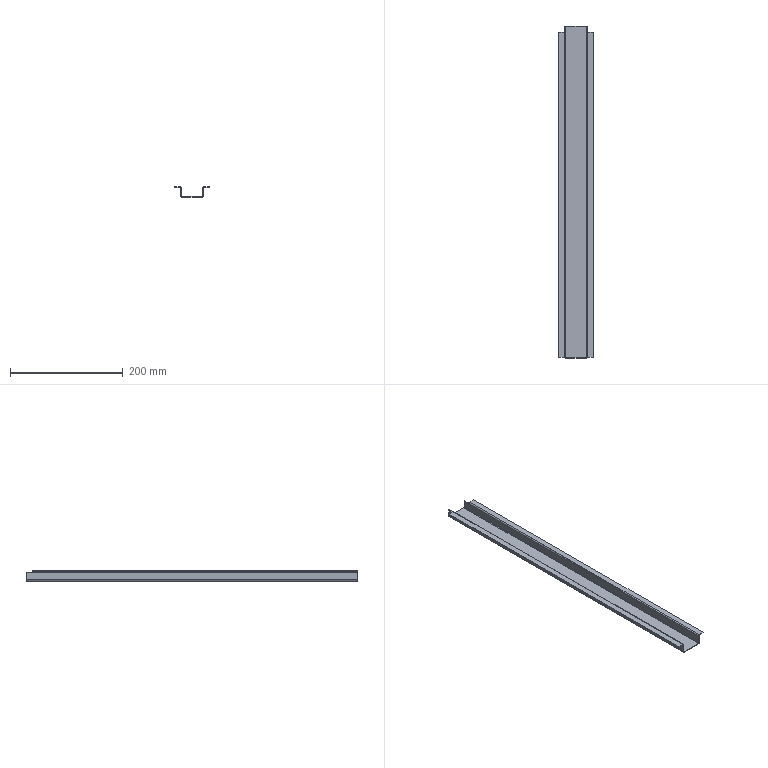Component | SolidWorks | AirFurnaceElectricalCabinet-DoorPanelAssembly-1_DoorPanelReinforcementPlate-L590-1 | 1 solid | 38 faces | box 61.6 x 590 x 18 mm | volume 65385 mm3 | plane 30 | cylinder 8 | commonest cylinder face diameters 3.9 x4 1.5 x4
STEP:
#1=COLOUR_RGB('',0.7922,0.8196,0.9333);
#2=FILL_AREA_STYLE_COLOUR('',#1);
#3=FILL_AREA_STYLE('',(#2));
#4=SURFACE_STYLE_FILL_AREA(#3);
#5=SURFACE_SIDE_STYLE('',(#4));
#6=SURFACE_STYLE_USAGE(.BOTH.,#5);
#7=PRESENTATION_STYLE_ASSIGNMENT((#6));
#8=CARTESIAN_POINT('',(0.7402,27.303,9.348));
#9=VERTEX_POINT('',#8);
#10=CARTESIAN_POINT('',(0.7402,27.303,9.882));
#11=VERTEX_POINT('',#10);
#12=CARTESIAN_POINT('',(0.7402,27.303,9.272));
#13=DIRECTION('',(-0.,-0.,1.));
#14=VECTOR('',#13,39.37);
#15=LINE('',#12,#14);
#16=EDGE_CURVE('',#9,#11,#15,.T.);
#17=ORIENTED_EDGE('',*,*,#16,.T.);
#18=CARTESIAN_POINT('',(0.7874,27.303,9.882));
#19=VERTEX_POINT('',#18);
#20=CARTESIAN_POINT('',(0.7106,27.303,9.882));
#21=DIRECTION('',(1.,-0.,0.));
#22=VECTOR('',#21,39.37);
#23=LINE('',#20,#22);
#24=EDGE_CURVE('',#11,#19,#23,.T.);
#25=ORIENTED_EDGE('',*,*,#24,.T.);
#26=CARTESIAN_POINT('',(0.7874,27.303,9.348));
#27=VERTEX_POINT('',#26);
#28=CARTESIAN_POINT('',(0.7874,27.303,9.272));
#29=DIRECTION('',(-0.,-0.,1.));
#30=VECTOR('',#29,39.37);
#31=LINE('',#28,#30);
#32=EDGE_CURVE('',#27,#19,#31,.T.);
#33=ORIENTED_EDGE('',*,*,#32,.F.);
#34=CARTESIAN_POINT('',(0.7874,27.303,9.348));
#35=DIRECTION('',(-1.,0.,-0.));
#36=VECTOR('',#35,39.37);
#37=LINE('',#34,#36);
#38=EDGE_CURVE('',#27,#9,#37,.T.);
#39=ORIENTED_EDGE('',*,*,#38,.T.);
#40=EDGE_LOOP('',(#17,#25,#33,#39));
#41=FACE_OUTER_BOUND('',#40,.T.);
#42=CARTESIAN_POINT('',(0.7106,27.303,9.319));
#43=DIRECTION('',(0.,1.,0.));
#44=DIRECTION('',(1.,-0.,0.));
#45=AXIS2_PLACEMENT_3D('',#42,#43,#44);
#46=PLANE('',#45);
#47=ADVANCED_FACE('',(#41),#46,.T.);
#48=CARTESIAN_POINT('',(0.7874,4.075,9.348));
#49=VERTEX_POINT('',#48);
#50=CARTESIAN_POINT('',(0.7874,4.075,9.882));
#51=VERTEX_POINT('',#50);
#52=CARTESIAN_POINT('',(0.7874,4.075,9.272));
#53=DIRECTION('',(-0.,-0.,1.));
#54=VECTOR('',#53,39.37);
#55=LINE('',#52,#54);
#56=EDGE_CURVE('',#49,#51,#55,.T.);
#57=ORIENTED_EDGE('',*,*,#56,.T.);
#58=CARTESIAN_POINT('',(0.7402,4.075,9.882));
#59=VERTEX_POINT('',#58);
#60=CARTESIAN_POINT('',(0.8169,4.075,9.882));
#61=DIRECTION('',(-1.,0.,-0.));
#62=VECTOR('',#61,39.37);
#63=LINE('',#60,#62);
#64=EDGE_CURVE('',#51,#59,#63,.T.);
#65=ORIENTED_EDGE('',*,*,#64,.T.);
#66=CARTESIAN_POINT('',(0.7402,4.075,9.348));
#67=VERTEX_POINT('',#66);
#68=CARTESIAN_POINT('',(0.7402,4.075,9.272));
#69=DIRECTION('',(-0.,-0.,1.));
#70=VECTOR('',#69,39.37);
#71=LINE('',#68,#70);
#72=EDGE_CURVE('',#67,#59,#71,.T.);
#73=ORIENTED_EDGE('',*,*,#72,.F.);
#74=CARTESIAN_POINT('',(0.7402,4.075,9.348));
#75=DIRECTION('',(1.,-0.,0.));
#76=VECTOR('',#75,39.37);
#77=LINE('',#74,#76);
#78=EDGE_CURVE('',#67,#49,#77,.T.);
#79=ORIENTED_EDGE('',*,*,#78,.T.);
#80=EDGE_LOOP('',(#57,#65,#73,#79));
#81=FACE_OUTER_BOUND('',#80,.T.);
#82=CARTESIAN_POINT('',(0.8169,4.075,9.98));
#83=DIRECTION('',(-0.,-1.,-0.));
#84=DIRECTION('',(-1.,0.,-0.));
#85=AXIS2_PLACEMENT_3D('',#82,#83,#84);
#86=PLANE('',#85);
#87=ADVANCED_FACE('',(#81),#86,.T.);
#88=CARTESIAN_POINT('',(-0.7402,4.075,9.882));
#89=VERTEX_POINT('',#88);
#90=CARTESIAN_POINT('',(-0.7402,4.075,9.348));
#91=VERTEX_POINT('',#90);
#92=CARTESIAN_POINT('',(-0.7402,4.075,9.933));
#93=DIRECTION('',(0.,0.,-1.));
#94=VECTOR('',#93,39.37);
#95=LINE('',#92,#94);
#96=EDGE_CURVE('',#89,#91,#95,.T.);
#97=ORIENTED_EDGE('',*,*,#96,.F.);
#98=CARTESIAN_POINT('',(-0.7874,4.075,9.882));
#99=VERTEX_POINT('',#98);
#100=CARTESIAN_POINT('',(-0.7106,4.075,9.882));
#101=DIRECTION('',(-1.,0.,-0.));
#102=VECTOR('',#101,39.37);
#103=LINE('',#100,#102);
#104=EDGE_CURVE('',#89,#99,#103,.T.);
#105=ORIENTED_EDGE('',*,*,#104,.T.);
#106=CARTESIAN_POINT('',(-0.7874,4.075,9.348));
#107=VERTEX_POINT('',#106);
#108=CARTESIAN_POINT('',(-0.7874,4.075,9.933));
#109=DIRECTION('',(0.,0.,-1.));
#110=VECTOR('',#109,39.37);
#111=LINE('',#108,#110);
#112=EDGE_CURVE('',#99,#107,#111,.T.);
#113=ORIENTED_EDGE('',*,*,#112,.T.);
#114=CARTESIAN_POINT('',(-0.7874,4.075,9.348));
#115=DIRECTION('',(1.,-0.,0.));
#116=VECTOR('',#115,39.37);
#117=LINE('',#114,#116);
#118=EDGE_CURVE('',#107,#91,#117,.T.);
#119=ORIENTED_EDGE('',*,*,#118,.T.);
#120=EDGE_LOOP('',(#97,#105,#113,#119));
#121=FACE_OUTER_BOUND('',#120,.T.);
#122=CARTESIAN_POINT('',(-0.7106,4.075,9.319));
#123=DIRECTION('',(-0.,-1.,-0.));
#124=DIRECTION('',(-1.,0.,-0.));
#125=AXIS2_PLACEMENT_3D('',#122,#123,#124);
#126=PLANE('',#125);
#127=ADVANCED_FACE('',(#121),#126,.T.);
#128=CARTESIAN_POINT('',(-0.7874,27.303,9.882));
#129=VERTEX_POINT('',#128);
#130=CARTESIAN_POINT('',(-0.7874,27.303,9.348));
#131=VERTEX_POINT('',#130);
#132=CARTESIAN_POINT('',(-0.7874,27.303,9.933));
#133=DIRECTION('',(0.,0.,-1.));
#134=VECTOR('',#133,39.37);
#135=LINE('',#132,#134);
#136=EDGE_CURVE('',#129,#131,#135,.T.);
#137=ORIENTED_EDGE('',*,*,#136,.F.);
#138=CARTESIAN_POINT('',(-0.7402,27.303,9.882));
#139=VERTEX_POINT('',#138);
#140=CARTESIAN_POINT('',(-0.8169,27.303,9.882));
#141=DIRECTION('',(1.,-0.,0.));
#142=VECTOR('',#141,39.37);
#143=LINE('',#140,#142);
#144=EDGE_CURVE('',#129,#139,#143,.T.);
#145=ORIENTED_EDGE('',*,*,#144,.T.);
#146=CARTESIAN_POINT('',(-0.7402,27.303,9.348));
#147=VERTEX_POINT('',#146);
#148=CARTESIAN_POINT('',(-0.7402,27.303,9.933));
#149=DIRECTION('',(0.,0.,-1.));
#150=VECTOR('',#149,39.37);
#151=LINE('',#148,#150);
#152=EDGE_CURVE('',#139,#147,#151,.T.);
#153=ORIENTED_EDGE('',*,*,#152,.T.);
#154=CARTESIAN_POINT('',(-0.7402,27.303,9.348));
#155=DIRECTION('',(-1.,0.,-0.));
#156=VECTOR('',#155,39.37);
#157=LINE('',#154,#156);
#158=EDGE_CURVE('',#147,#131,#157,.T.);
#159=ORIENTED_EDGE('',*,*,#158,.T.);
#160=EDGE_LOOP('',(#137,#145,#153,#159));
#161=FACE_OUTER_BOUND('',#160,.T.);
#162=CARTESIAN_POINT('',(-0.8169,27.303,9.98));
#163=DIRECTION('',(0.,1.,0.));
#164=DIRECTION('',(1.,-0.,0.));
#165=AXIS2_PLACEMENT_3D('',#162,#163,#164);
#166=PLANE('',#165);
#167=ADVANCED_FACE('',(#161),#166,.T.);
#168=CARTESIAN_POINT('',(-0.7106,27.303,9.272));
#169=VERTEX_POINT('',#168);
#170=CARTESIAN_POINT('',(0.7106,27.303,9.272));
#171=VERTEX_POINT('',#170);
#172=CARTESIAN_POINT('',(-0.7874,27.303,9.272));
#173=DIRECTION('',(1.,-0.,0.));
#174=VECTOR('',#173,39.37);
#175=LINE('',#172,#174);
#176=EDGE_CURVE('',#169,#171,#175,.T.);
#177=ORIENTED_EDGE('',*,*,#176,.F.);
#178=CARTESIAN_POINT('',(-0.7106,27.303,9.319));
#179=VERTEX_POINT('',#178);
#180=CARTESIAN_POINT('',(-0.7106,27.303,9.272));
#181=DIRECTION('',(-0.,-0.,1.));
#182=VECTOR('',#181,39.37);
#183=LINE('',#180,#182);
#184=EDGE_CURVE('',#169,#179,#183,.T.);
#185=ORIENTED_EDGE('',*,*,#184,.T.);
#186=CARTESIAN_POINT('',(0.7106,27.303,9.319));
#187=VERTEX_POINT('',#186);
#188=CARTESIAN_POINT('',(-0.7874,27.303,9.319));
#189=DIRECTION('',(1.,-0.,0.));
#190=VECTOR('',#189,39.37);
#191=LINE('',#188,#190);
#192=EDGE_CURVE('',#179,#187,#191,.T.);
#193=ORIENTED_EDGE('',*,*,#192,.T.);
#194=CARTESIAN_POINT('',(0.7106,27.303,9.319));
#195=DIRECTION('',(0.,0.,-1.));
#196=VECTOR('',#195,39.37);
#197=LINE('',#194,#196);
#198=EDGE_CURVE('',#187,#171,#197,.T.);
#199=ORIENTED_EDGE('',*,*,#198,.T.);
#200=EDGE_LOOP('',(#177,#185,#193,#199));
#201=FACE_OUTER_BOUND('',#200,.T.);
#202=CARTESIAN_POINT('',(-0.7402,27.303,9.348));
#203=DIRECTION('',(0.,1.,0.));
#204=DIRECTION('',(1.,-0.,0.));
#205=AXIS2_PLACEMENT_3D('',#202,#203,#204);
#206=PLANE('',#205);
#207=ADVANCED_FACE('',(#201),#206,.T.);
#208=CARTESIAN_POINT('',(-0.7106,4.075,9.272));
#209=VERTEX_POINT('',#208);
#210=CARTESIAN_POINT('',(0.7106,4.075,9.272));
#211=VERTEX_POINT('',#210);
#212=CARTESIAN_POINT('',(-0.7874,4.075,9.272));
#213=DIRECTION('',(1.,-0.,0.));
#214=VECTOR('',#213,39.37);
#215=LINE('',#212,#214);
#216=EDGE_CURVE('',#209,#211,#215,.T.);
#217=ORIENTED_EDGE('',*,*,#216,.T.);
#218=CARTESIAN_POINT('',(0.7106,4.075,9.319));
#219=VERTEX_POINT('',#218);
#220=CARTESIAN_POINT('',(0.7106,4.075,9.272));
#221=DIRECTION('',(-0.,-0.,1.));
#222=VECTOR('',#221,39.37);
#223=LINE('',#220,#222);
#224=EDGE_CURVE('',#211,#219,#223,.T.);
#225=ORIENTED_EDGE('',*,*,#224,.T.);
#226=CARTESIAN_POINT('',(-0.7106,4.075,9.319));
#227=VERTEX_POINT('',#226);
#228=CARTESIAN_POINT('',(-0.7874,4.075,9.319));
#229=DIRECTION('',(1.,-0.,0.));
#230=VECTOR('',#229,39.37);
#231=LINE('',#228,#230);
#232=EDGE_CURVE('',#227,#219,#231,.T.);
#233=ORIENTED_EDGE('',*,*,#232,.F.);
#234=CARTESIAN_POINT('',(-0.7106,4.075,9.319));
#235=DIRECTION('',(0.,0.,-1.));
#236=VECTOR('',#235,39.37);
#237=LINE('',#234,#236);
#238=EDGE_CURVE('',#227,#209,#237,.T.);
#239=ORIENTED_EDGE('',*,*,#238,.T.);
#240=EDGE_LOOP('',(#217,#225,#233,#239));
#241=FACE_OUTER_BOUND('',#240,.T.);
#242=CARTESIAN_POINT('',(0.7402,4.075,9.348));
#243=DIRECTION('',(-0.,-1.,-0.));
#244=DIRECTION('',(-1.,0.,-0.));
#245=AXIS2_PLACEMENT_3D('',#242,#243,#244);
#246=PLANE('',#245);
#247=ADVANCED_FACE('',(#241),#246,.T.);
#248=ORIENTED_EDGE('',*,*,#216,.F.);
#249=CARTESIAN_POINT('',(-0.7106,27.303,9.272));
#250=DIRECTION('',(-0.,-1.,-0.));
#251=VECTOR('',#250,39.37);
#252=LINE('',#249,#251);
#253=EDGE_CURVE('',#169,#209,#252,.T.);
#254=ORIENTED_EDGE('',*,*,#253,.F.);
#255=ORIENTED_EDGE('',*,*,#176,.T.);
#256=CARTESIAN_POINT('',(0.7106,27.303,9.272));
#257=DIRECTION('',(-0.,-1.,-0.));
#258=VECTOR('',#257,39.37);
#259=LINE('',#256,#258);
#260=EDGE_CURVE('',#171,#211,#259,.T.);
#261=ORIENTED_EDGE('',*,*,#260,.T.);
#262=EDGE_LOOP('',(#248,#254,#255,#261));
#263=FACE_OUTER_BOUND('',#262,.T.);
#264=CARTESIAN_POINT('',(-0.7874,27.303,9.272));
#265=DIRECTION('',(0.,0.,-1.));
#266=DIRECTION('',(-1.,0.,-0.));
#267=AXIS2_PLACEMENT_3D('',#264,#265,#266);
#268=PLANE('',#267);
#269=ADVANCED_FACE('',(#263),#268,.T.);
#270=ORIENTED_EDGE('',*,*,#232,.T.);
#271=CARTESIAN_POINT('',(0.7106,27.303,9.319));
#272=DIRECTION('',(-0.,-1.,-0.));
#273=VECTOR('',#272,39.37);
#274=LINE('',#271,#273);
#275=EDGE_CURVE('',#187,#219,#274,.T.);
#276=ORIENTED_EDGE('',*,*,#275,.F.);
#277=ORIENTED_EDGE('',*,*,#192,.F.);
#278=CARTESIAN_POINT('',(-0.7106,27.303,9.319));
#279=DIRECTION('',(-0.,-1.,-0.));
#280=VECTOR('',#279,39.37);
#281=LINE('',#278,#280);
#282=EDGE_CURVE('',#179,#227,#281,.T.);
#283=ORIENTED_EDGE('',*,*,#282,.T.);
#284=EDGE_LOOP('',(#270,#276,#277,#283));
#285=FACE_OUTER_BOUND('',#284,.T.);
#286=CARTESIAN_POINT('',(-0.7874,27.303,9.319));
#287=DIRECTION('',(0.,0.,-1.));
#288=DIRECTION('',(-1.,0.,-0.));
#289=AXIS2_PLACEMENT_3D('',#286,#287,#288);
#290=PLANE('',#289);
#291=ADVANCED_FACE('',(#285),#290,.F.);
#292=ORIENTED_EDGE('',*,*,#198,.F.);
#293=CARTESIAN_POINT('',(0.7106,27.303,9.348));
#294=DIRECTION('',(-0.,-1.,-0.));
#295=DIRECTION('',(-1.,0.,0.));
#296=AXIS2_PLACEMENT_3D('',#293,#294,#295);
#297=CIRCLE('',#296,0.02953);
#298=EDGE_CURVE('',#187,#9,#297,.T.);
#299=ORIENTED_EDGE('',*,*,#298,.T.);
#300=ORIENTED_EDGE('',*,*,#38,.F.);
#301=CARTESIAN_POINT('',(0.7106,27.303,9.348));
#302=DIRECTION('',(-0.,-1.,-0.));
#303=DIRECTION('',(-1.,0.,0.));
#304=AXIS2_PLACEMENT_3D('',#301,#302,#303);
#305=CIRCLE('',#304,0.07677);
#306=EDGE_CURVE('',#171,#27,#305,.T.);
#307=ORIENTED_EDGE('',*,*,#306,.F.);
#308=EDGE_LOOP('',(#292,#299,#300,#307));
#309=FACE_OUTER_BOUND('',#308,.T.);
#310=CARTESIAN_POINT('',(0.7106,27.303,9.348));
#311=DIRECTION('',(0.,1.,0.));
#312=DIRECTION('',(1.,-0.,0.));
#313=AXIS2_PLACEMENT_3D('',#310,#311,#312);
#314=PLANE('',#313);
#315=ADVANCED_FACE('',(#309),#314,.T.);
#316=ORIENTED_EDGE('',*,*,#78,.F.);
#317=CARTESIAN_POINT('',(0.7106,4.075,9.348));
#318=DIRECTION('',(0.,1.,0.));
#319=DIRECTION('',(-1.,0.,0.));
#320=AXIS2_PLACEMENT_3D('',#317,#318,#319);
#321=CIRCLE('',#320,0.02953);
#322=EDGE_CURVE('',#67,#219,#321,.T.);
#323=ORIENTED_EDGE('',*,*,#322,.T.);
#324=ORIENTED_EDGE('',*,*,#224,.F.);
#325=CARTESIAN_POINT('',(0.7106,4.075,9.348));
#326=DIRECTION('',(0.,1.,0.));
#327=DIRECTION('',(1.,0.,0.));
#328=AXIS2_PLACEMENT_3D('',#325,#326,#327);
#329=CIRCLE('',#328,0.07677);
#330=EDGE_CURVE('',#49,#211,#329,.T.);
#331=ORIENTED_EDGE('',*,*,#330,.F.);
#332=EDGE_LOOP('',(#316,#323,#324,#331));
#333=FACE_OUTER_BOUND('',#332,.T.);
#334=CARTESIAN_POINT('',(0.7106,4.075,9.348));
#335=DIRECTION('',(-0.,-1.,-0.));
#336=DIRECTION('',(-1.,0.,-0.));
#337=AXIS2_PLACEMENT_3D('',#334,#335,#336);
#338=PLANE('',#337);
#339=ADVANCED_FACE('',(#333),#338,.T.);
#340=ORIENTED_EDGE('',*,*,#330,.T.);
#341=ORIENTED_EDGE('',*,*,#260,.F.);
#342=ORIENTED_EDGE('',*,*,#306,.T.);
#343=CARTESIAN_POINT('',(0.7874,27.303,9.348));
#344=DIRECTION('',(-0.,-1.,-0.));
#345=VECTOR('',#344,39.37);
#346=LINE('',#343,#345);
#347=EDGE_CURVE('',#27,#49,#346,.T.);
#348=ORIENTED_EDGE('',*,*,#347,.T.);
#349=EDGE_LOOP('',(#340,#341,#342,#348));
#350=FACE_OUTER_BOUND('',#349,.T.);
#351=CARTESIAN_POINT('',(0.7106,38.917,9.348));
#352=DIRECTION('',(-0.,-1.,-0.));
#353=DIRECTION('',(-1.,0.,0.));
#354=AXIS2_PLACEMENT_3D('',#351,#352,#353);
#355=CYLINDRICAL_SURFACE('',#354,0.07677);
#356=ADVANCED_FACE('',(#350),#355,.T.);
#357=ORIENTED_EDGE('',*,*,#322,.F.);
#358=CARTESIAN_POINT('',(0.7402,27.303,9.348));
#359=DIRECTION('',(-0.,-1.,-0.));
#360=VECTOR('',#359,39.37);
#361=LINE('',#358,#360);
#362=EDGE_CURVE('',#9,#67,#361,.T.);
#363=ORIENTED_EDGE('',*,*,#362,.F.);
#364=ORIENTED_EDGE('',*,*,#298,.F.);
#365=ORIENTED_EDGE('',*,*,#275,.T.);
#366=EDGE_LOOP('',(#357,#363,#364,#365));
#367=FACE_OUTER_BOUND('',#366,.T.);
#368=CARTESIAN_POINT('',(0.7106,38.917,9.348));
#369=DIRECTION('',(-0.,-1.,-0.));
#370=DIRECTION('',(-1.,0.,0.));
#371=AXIS2_PLACEMENT_3D('',#368,#369,#370);
#372=CYLINDRICAL_SURFACE('',#371,0.02953);
#373=ADVANCED_FACE('',(#367),#372,.F.);
#374=CARTESIAN_POINT('',(1.213,4.114,9.933));
#375=VERTEX_POINT('',#374);
#376=CARTESIAN_POINT('',(1.213,4.114,9.98));
#377=VERTEX_POINT('',#376);
#378=CARTESIAN_POINT('',(1.213,4.114,9.933));
#379=DIRECTION('',(-0.,-0.,1.));
#380=VECTOR('',#379,39.37);
#381=LINE('',#378,#380);
#382=EDGE_CURVE('',#375,#377,#381,.T.);
#383=ORIENTED_EDGE('',*,*,#382,.F.);
#384=CARTESIAN_POINT('',(1.213,26.858,9.933));
#385=VERTEX_POINT('',#384);
#386=CARTESIAN_POINT('',(1.213,27.303,9.933));
#387=DIRECTION('',(-0.,-1.,-0.));
#388=VECTOR('',#387,39.37);
#389=LINE('',#386,#388);
#390=EDGE_CURVE('',#385,#375,#389,.T.);
#391=ORIENTED_EDGE('',*,*,#390,.F.);
#392=CARTESIAN_POINT('',(1.213,26.858,9.98));
#393=VERTEX_POINT('',#392);
#394=CARTESIAN_POINT('',(1.213,26.858,9.933));
#395=DIRECTION('',(0.,0.,-1.));
#396=VECTOR('',#395,39.37);
#397=LINE('',#394,#396);
#398=EDGE_CURVE('',#393,#385,#397,.T.);
#399=ORIENTED_EDGE('',*,*,#398,.F.);
#400=CARTESIAN_POINT('',(1.213,27.303,9.98));
#401=DIRECTION('',(-0.,-1.,-0.));
#402=VECTOR('',#401,39.37);
#403=LINE('',#400,#402);
#404=EDGE_CURVE('',#393,#377,#403,.T.);
#405=ORIENTED_EDGE('',*,*,#404,.T.);
#406=EDGE_LOOP('',(#383,#391,#399,#405));
#407=FACE_OUTER_BOUND('',#406,.T.);
#408=CARTESIAN_POINT('',(1.213,27.303,9.933));
#409=DIRECTION('',(1.,-0.,0.));
#410=DIRECTION('',(-0.,-1.,-0.));
#411=AXIS2_PLACEMENT_3D('',#408,#409,#410);
#412=PLANE('',#411);
#413=ADVANCED_FACE('',(#407),#412,.T.);
#414=CARTESIAN_POINT('',(0.8169,26.858,9.98));
#415=VERTEX_POINT('',#414);
#416=CARTESIAN_POINT('',(0.8169,4.114,9.98));
#417=VERTEX_POINT('',#416);
#418=CARTESIAN_POINT('',(0.8169,27.303,9.98));
#419=DIRECTION('',(-0.,-1.,-0.));
#420=VECTOR('',#419,39.37);
#421=LINE('',#418,#420);
#422=EDGE_CURVE('',#415,#417,#421,.T.);
#423=ORIENTED_EDGE('',*,*,#422,.T.);
#424=CARTESIAN_POINT('',(0.7874,4.114,9.98));
#425=DIRECTION('',(1.,-0.,0.));
#426=VECTOR('',#425,39.37);
#427=LINE('',#424,#426);
#428=EDGE_CURVE('',#417,#377,#427,.T.);
#429=ORIENTED_EDGE('',*,*,#428,.T.);
#430=ORIENTED_EDGE('',*,*,#404,.F.);
#431=CARTESIAN_POINT('',(0.7874,26.858,9.98));
#432=DIRECTION('',(-1.,0.,-0.));
#433=VECTOR('',#432,39.37);
#434=LINE('',#431,#433);
#435=EDGE_CURVE('',#393,#415,#434,.T.);
#436=ORIENTED_EDGE('',*,*,#435,.T.);
#437=EDGE_LOOP('',(#423,#429,#430,#436));
#438=FACE_OUTER_BOUND('',#437,.T.);
#439=CARTESIAN_POINT('',(0.7874,27.303,9.98));
#440=DIRECTION('',(0.,0.,-1.));
#441=DIRECTION('',(-1.,0.,-0.));
#442=AXIS2_PLACEMENT_3D('',#439,#440,#441);
#443=PLANE('',#442);
#444=ADVANCED_FACE('',(#438),#443,.F.);
#445=CARTESIAN_POINT('',(0.8169,4.114,9.933));
#446=VERTEX_POINT('',#445);
#447=CARTESIAN_POINT('',(0.7874,4.114,9.933));
#448=DIRECTION('',(1.,-0.,0.));
#449=VECTOR('',#448,39.37);
#450=LINE('',#447,#449);
#451=EDGE_CURVE('',#446,#375,#450,.T.);
#452=ORIENTED_EDGE('',*,*,#451,.F.);
#453=CARTESIAN_POINT('',(0.8169,26.858,9.933));
#454=VERTEX_POINT('',#453);
#455=CARTESIAN_POINT('',(0.8169,27.303,9.933));
#456=DIRECTION('',(-0.,-1.,-0.));
#457=VECTOR('',#456,39.37);
#458=LINE('',#455,#457);
#459=EDGE_CURVE('',#454,#446,#458,.T.);
#460=ORIENTED_EDGE('',*,*,#459,.F.);
#461=CARTESIAN_POINT('',(0.7874,26.858,9.933));
#462=DIRECTION('',(-1.,0.,-0.));
#463=VECTOR('',#462,39.37);
#464=LINE('',#461,#463);
#465=EDGE_CURVE('',#385,#454,#464,.T.);
#466=ORIENTED_EDGE('',*,*,#465,.F.);
#467=ORIENTED_EDGE('',*,*,#390,.T.);
#468=EDGE_LOOP('',(#452,#460,#466,#467));
#469=FACE_OUTER_BOUND('',#468,.T.);
#470=CARTESIAN_POINT('',(0.7874,27.303,9.933));
#471=DIRECTION('',(0.,0.,-1.));
#472=DIRECTION('',(-1.,0.,-0.));
#473=AXIS2_PLACEMENT_3D('',#470,#471,#472);
#474=PLANE('',#473);
#475=ADVANCED_FACE('',(#469),#474,.T.);
#476=CARTESIAN_POINT('',(0.7402,26.858,9.904));
#477=VERTEX_POINT('',#476);
#478=CARTESIAN_POINT('',(0.7402,4.114,9.904));
#479=VERTEX_POINT('',#478);
#480=CARTESIAN_POINT('',(0.7402,27.303,9.904));
#481=DIRECTION('',(-0.,-1.,-0.));
#482=VECTOR('',#481,39.37);
#483=LINE('',#480,#482);
#484=EDGE_CURVE('',#477,#479,#483,.T.);
#485=ORIENTED_EDGE('',*,*,#484,.T.);
#486=CARTESIAN_POINT('',(0.8169,4.114,9.904));
#487=DIRECTION('',(0.,1.,0.));
#488=DIRECTION('',(1.,0.,0.));
#489=AXIS2_PLACEMENT_3D('',#486,#487,#488);
#490=CIRCLE('',#489,0.07677);
#491=EDGE_CURVE('',#479,#417,#490,.T.);
#492=ORIENTED_EDGE('',*,*,#491,.T.);
#493=ORIENTED_EDGE('',*,*,#422,.F.);
#494=CARTESIAN_POINT('',(0.8169,26.858,9.904));
#495=DIRECTION('',(-0.,-1.,-0.));
#496=DIRECTION('',(-1.,0.,0.));
#497=AXIS2_PLACEMENT_3D('',#494,#495,#496);
#498=CIRCLE('',#497,0.07677);
#499=EDGE_CURVE('',#415,#477,#498,.T.);
#500=ORIENTED_EDGE('',*,*,#499,.T.);
#501=EDGE_LOOP('',(#485,#492,#493,#500));
#502=FACE_OUTER_BOUND('',#501,.T.);
#503=CARTESIAN_POINT('',(0.8169,38.917,9.904));
#504=DIRECTION('',(-0.,-1.,-0.));
#505=DIRECTION('',(0.,0.,-1.));
#506=AXIS2_PLACEMENT_3D('',#503,#504,#505);
#507=CYLINDRICAL_SURFACE('',#506,0.07677);
#508=ADVANCED_FACE('',(#502),#507,.T.);
#509=CARTESIAN_POINT('',(0.7874,4.114,9.904));
#510=VERTEX_POINT('',#509);
#511=CARTESIAN_POINT('',(0.8169,4.114,9.904));
#512=DIRECTION('',(0.,1.,0.));
#513=DIRECTION('',(1.,0.,0.));
#514=AXIS2_PLACEMENT_3D('',#511,#512,#513);
#515=CIRCLE('',#514,0.02953);
#516=EDGE_CURVE('',#510,#446,#515,.T.);
#517=ORIENTED_EDGE('',*,*,#516,.F.);
#518=CARTESIAN_POINT('',(0.7874,26.858,9.904));
#519=VERTEX_POINT('',#518);
#520=CARTESIAN_POINT('',(0.7874,27.303,9.904));
#521=DIRECTION('',(-0.,-1.,-0.));
#522=VECTOR('',#521,39.37);
#523=LINE('',#520,#522);
#524=EDGE_CURVE('',#519,#510,#523,.T.);
#525=ORIENTED_EDGE('',*,*,#524,.F.);
#526=CARTESIAN_POINT('',(0.8169,26.858,9.904));
#527=DIRECTION('',(-0.,-1.,-0.));
#528=DIRECTION('',(-1.,0.,0.));
#529=AXIS2_PLACEMENT_3D('',#526,#527,#528);
#530=CIRCLE('',#529,0.02953);
#531=EDGE_CURVE('',#454,#519,#530,.T.);
#532=ORIENTED_EDGE('',*,*,#531,.F.);
#533=ORIENTED_EDGE('',*,*,#459,.T.);
#534=EDGE_LOOP('',(#517,#525,#532,#533));
#535=FACE_OUTER_BOUND('',#534,.T.);
#536=CARTESIAN_POINT('',(0.8169,38.917,9.904));
#537=DIRECTION('',(-0.,-1.,-0.));
#538=DIRECTION('',(0.,0.,-1.));
#539=AXIS2_PLACEMENT_3D('',#536,#537,#538);
#540=CYLINDRICAL_SURFACE('',#539,0.02953);
#541=ADVANCED_FACE('',(#535),#540,.F.);
#542=CARTESIAN_POINT('',(0.7874,4.114,9.882));
#543=VERTEX_POINT('',#542);
#544=CARTESIAN_POINT('',(0.7874,4.114,9.272));
#545=DIRECTION('',(-0.,-0.,1.));
#546=VECTOR('',#545,39.37);
#547=LINE('',#544,#546);
#548=EDGE_CURVE('',#543,#510,#547,.T.);
#549=ORIENTED_EDGE('',*,*,#548,.F.);
#550=CARTESIAN_POINT('',(0.7874,27.303,9.882));
#551=DIRECTION('',(-0.,-1.,-0.));
#552=VECTOR('',#551,39.37);
#553=LINE('',#550,#552);
#554=EDGE_CURVE('',#543,#51,#553,.T.);
#555=ORIENTED_EDGE('',*,*,#554,.T.);
#556=ORIENTED_EDGE('',*,*,#56,.F.);
#557=ORIENTED_EDGE('',*,*,#347,.F.);
#558=ORIENTED_EDGE('',*,*,#32,.T.);
#559=CARTESIAN_POINT('',(0.7874,26.858,9.882));
#560=VERTEX_POINT('',#559);
#561=CARTESIAN_POINT('',(0.7874,27.303,9.882));
#562=DIRECTION('',(-0.,-1.,-0.));
#563=VECTOR('',#562,39.37);
#564=LINE('',#561,#563);
#565=EDGE_CURVE('',#19,#560,#564,.T.);
#566=ORIENTED_EDGE('',*,*,#565,.T.);
#567=CARTESIAN_POINT('',(0.7874,26.858,9.272));
#568=DIRECTION('',(0.,0.,-1.));
#569=VECTOR('',#568,39.37);
#570=LINE('',#567,#569);
#571=EDGE_CURVE('',#519,#560,#570,.T.);
#572=ORIENTED_EDGE('',*,*,#571,.F.);
#573=ORIENTED_EDGE('',*,*,#524,.T.);
#574=EDGE_LOOP('',(#549,#555,#556,#557,#558,#566,#572,#573));
#575=FACE_OUTER_BOUND('',#574,.T.);
#576=CARTESIAN_POINT('',(0.7874,27.303,9.272));
#577=DIRECTION('',(1.,-0.,0.));
#578=DIRECTION('',(-0.,-1.,-0.));
#579=AXIS2_PLACEMENT_3D('',#576,#577,#578);
#580=PLANE('',#579);
#581=ADVANCED_FACE('',(#575),#580,.T.);
#582=CARTESIAN_POINT('',(0.7402,4.114,9.882));
#583=VERTEX_POINT('',#582);
#584=CARTESIAN_POINT('',(0.7402,27.303,9.882));
#585=DIRECTION('',(-0.,-1.,-0.));
#586=VECTOR('',#585,39.37);
#587=LINE('',#584,#586);
#588=EDGE_CURVE('',#583,#59,#587,.T.);
#589=ORIENTED_EDGE('',*,*,#588,.F.);
#590=CARTESIAN_POINT('',(0.7402,4.114,9.272));
#591=DIRECTION('',(-0.,-0.,1.));
#592=VECTOR('',#591,39.37);
#593=LINE('',#590,#592);
#594=EDGE_CURVE('',#583,#479,#593,.T.);
#595=ORIENTED_EDGE('',*,*,#594,.T.);
#596=ORIENTED_EDGE('',*,*,#484,.F.);
#597=CARTESIAN_POINT('',(0.7402,26.858,9.882));
#598=VERTEX_POINT('',#597);
#599=CARTESIAN_POINT('',(0.7402,26.858,9.272));
#600=DIRECTION('',(0.,0.,-1.));
#601=VECTOR('',#600,39.37);
#602=LINE('',#599,#601);
#603=EDGE_CURVE('',#477,#598,#602,.T.);
#604=ORIENTED_EDGE('',*,*,#603,.T.);
#605=CARTESIAN_POINT('',(0.7402,27.303,9.882));
#606=DIRECTION('',(-0.,-1.,-0.));
#607=VECTOR('',#606,39.37);
#608=LINE('',#605,#607);
#609=EDGE_CURVE('',#11,#598,#608,.T.);
#610=ORIENTED_EDGE('',*,*,#609,.F.);
#611=ORIENTED_EDGE('',*,*,#16,.F.);
#612=ORIENTED_EDGE('',*,*,#362,.T.);
#613=ORIENTED_EDGE('',*,*,#72,.T.);
#614=EDGE_LOOP('',(#589,#595,#596,#604,#610,#611,#612,#613));
#615=FACE_OUTER_BOUND('',#614,.T.);
#616=CARTESIAN_POINT('',(0.7402,27.303,9.272));
#617=DIRECTION('',(1.,-0.,0.));
#618=DIRECTION('',(-0.,-1.,-0.));
#619=AXIS2_PLACEMENT_3D('',#616,#617,#618);
#620=PLANE('',#619);
#621=ADVANCED_FACE('',(#615),#620,.F.);
#622=ORIENTED_EDGE('',*,*,#158,.F.);
#623=CARTESIAN_POINT('',(-0.7106,27.303,9.348));
#624=DIRECTION('',(-0.,-1.,-0.));
#625=DIRECTION('',(1.,0.,0.));
#626=AXIS2_PLACEMENT_3D('',#623,#624,#625);
#627=CIRCLE('',#626,0.02953);
#628=EDGE_CURVE('',#147,#179,#627,.T.);
#629=ORIENTED_EDGE('',*,*,#628,.T.);
#630=ORIENTED_EDGE('',*,*,#184,.F.);
#631=CARTESIAN_POINT('',(-0.7106,27.303,9.348));
#632=DIRECTION('',(-0.,-1.,-0.));
#633=DIRECTION('',(-1.,0.,0.));
#634=AXIS2_PLACEMENT_3D('',#631,#632,#633);
#635=CIRCLE('',#634,0.07677);
#636=EDGE_CURVE('',#131,#169,#635,.T.);
#637=ORIENTED_EDGE('',*,*,#636,.F.);
#638=EDGE_LOOP('',(#622,#629,#630,#637));
#639=FACE_OUTER_BOUND('',#638,.T.);
#640=CARTESIAN_POINT('',(-0.7106,27.303,9.348));
#641=DIRECTION('',(0.,1.,0.));
#642=DIRECTION('',(1.,-0.,0.));
#643=AXIS2_PLACEMENT_3D('',#640,#641,#642);
#644=PLANE('',#643);
#645=ADVANCED_FACE('',(#639),#644,.T.);
#646=ORIENTED_EDGE('',*,*,#238,.F.);
#647=CARTESIAN_POINT('',(-0.7106,4.075,9.348));
#648=DIRECTION('',(0.,1.,0.));
#649=DIRECTION('',(1.,0.,0.));
#650=AXIS2_PLACEMENT_3D('',#647,#648,#649);
#651=CIRCLE('',#650,0.02953);
#652=EDGE_CURVE('',#227,#91,#651,.T.);
#653=ORIENTED_EDGE('',*,*,#652,.T.);
#654=ORIENTED_EDGE('',*,*,#118,.F.);
#655=CARTESIAN_POINT('',(-0.7106,4.075,9.348));
#656=DIRECTION('',(0.,1.,0.));
#657=DIRECTION('',(1.,0.,0.));
#658=AXIS2_PLACEMENT_3D('',#655,#656,#657);
#659=CIRCLE('',#658,0.07677);
#660=EDGE_CURVE('',#209,#107,#659,.T.);
#661=ORIENTED_EDGE('',*,*,#660,.F.);
#662=EDGE_LOOP('',(#646,#653,#654,#661));
#663=FACE_OUTER_BOUND('',#662,.T.);
#664=CARTESIAN_POINT('',(-0.7106,4.075,9.348));
#665=DIRECTION('',(-0.,-1.,-0.));
#666=DIRECTION('',(-1.,0.,-0.));
#667=AXIS2_PLACEMENT_3D('',#664,#665,#666);
#668=PLANE('',#667);
#669=ADVANCED_FACE('',(#663),#668,.T.);
#670=ORIENTED_EDGE('',*,*,#660,.T.);
#671=CARTESIAN_POINT('',(-0.7874,27.303,9.348));
#672=DIRECTION('',(-0.,-1.,-0.));
#673=VECTOR('',#672,39.37);
#674=LINE('',#671,#673);
#675=EDGE_CURVE('',#131,#107,#674,.T.);
#676=ORIENTED_EDGE('',*,*,#675,.F.);
#677=ORIENTED_EDGE('',*,*,#636,.T.);
#678=ORIENTED_EDGE('',*,*,#253,.T.);
#679=EDGE_LOOP('',(#670,#676,#677,#678));
#680=FACE_OUTER_BOUND('',#679,.T.);
#681=CARTESIAN_POINT('',(-0.7106,-7.54,9.348));
#682=DIRECTION('',(0.,1.,0.));
#683=DIRECTION('',(1.,0.,0.));
#684=AXIS2_PLACEMENT_3D('',#681,#682,#683);
#685=CYLINDRICAL_SURFACE('',#684,0.07677);
#686=ADVANCED_FACE('',(#680),#685,.T.);
#687=ORIENTED_EDGE('',*,*,#652,.F.);
#688=ORIENTED_EDGE('',*,*,#282,.F.);
#689=ORIENTED_EDGE('',*,*,#628,.F.);
#690=CARTESIAN_POINT('',(-0.7402,27.303,9.348));
#691=DIRECTION('',(-0.,-1.,-0.));
#692=VECTOR('',#691,39.37);
#693=LINE('',#690,#692);
#694=EDGE_CURVE('',#147,#91,#693,.T.);
#695=ORIENTED_EDGE('',*,*,#694,.T.);
#696=EDGE_LOOP('',(#687,#688,#689,#695));
#697=FACE_OUTER_BOUND('',#696,.T.);
#698=CARTESIAN_POINT('',(-0.7106,-7.54,9.348));
#699=DIRECTION('',(0.,1.,0.));
#700=DIRECTION('',(1.,0.,0.));
#701=AXIS2_PLACEMENT_3D('',#698,#699,#700);
#702=CYLINDRICAL_SURFACE('',#701,0.02953);
#703=ADVANCED_FACE('',(#697),#702,.F.);
#704=CARTESIAN_POINT('',(-0.7874,4.114,9.904));
#705=VERTEX_POINT('',#704);
#706=CARTESIAN_POINT('',(-0.7874,4.114,9.882));
#707=VERTEX_POINT('',#706);
#708=CARTESIAN_POINT('',(-0.7874,4.114,9.933));
#709=DIRECTION('',(0.,0.,-1.));
#710=VECTOR('',#709,39.37);
#711=LINE('',#708,#710);
#712=EDGE_CURVE('',#705,#707,#711,.T.);
#713=ORIENTED_EDGE('',*,*,#712,.F.);
#714=CARTESIAN_POINT('',(-0.7874,26.858,9.904));
#715=VERTEX_POINT('',#714);
#716=CARTESIAN_POINT('',(-0.7874,27.303,9.904));
#717=DIRECTION('',(-0.,-1.,-0.));
#718=VECTOR('',#717,39.37);
#719=LINE('',#716,#718);
#720=EDGE_CURVE('',#715,#705,#719,.T.);
#721=ORIENTED_EDGE('',*,*,#720,.F.);
#722=CARTESIAN_POINT('',(-0.7874,26.858,9.882));
#723=VERTEX_POINT('',#722);
#724=CARTESIAN_POINT('',(-0.7874,26.858,9.933));
#725=DIRECTION('',(-0.,-0.,1.));
#726=VECTOR('',#725,39.37);
#727=LINE('',#724,#726);
#728=EDGE_CURVE('',#723,#715,#727,.T.);
#729=ORIENTED_EDGE('',*,*,#728,.F.);
#730=CARTESIAN_POINT('',(-0.7874,27.303,9.882));
#731=DIRECTION('',(0.,1.,0.));
#732=VECTOR('',#731,39.37);
#733=LINE('',#730,#732);
#734=EDGE_CURVE('',#723,#129,#733,.T.);
#735=ORIENTED_EDGE('',*,*,#734,.T.);
#736=ORIENTED_EDGE('',*,*,#136,.T.);
#737=ORIENTED_EDGE('',*,*,#675,.T.);
#738=ORIENTED_EDGE('',*,*,#112,.F.);
#739=CARTESIAN_POINT('',(-0.7874,27.303,9.882));
#740=DIRECTION('',(0.,1.,0.));
#741=VECTOR('',#740,39.37);
#742=LINE('',#739,#741);
#743=EDGE_CURVE('',#99,#707,#742,.T.);
#744=ORIENTED_EDGE('',*,*,#743,.T.);
#745=EDGE_LOOP('',(#713,#721,#729,#735,#736,#737,#738,#744));
#746=FACE_OUTER_BOUND('',#745,.T.);
#747=CARTESIAN_POINT('',(-0.7874,27.303,9.933));
#748=DIRECTION('',(-1.,0.,-0.));
#749=DIRECTION('',(0.,1.,0.));
#750=AXIS2_PLACEMENT_3D('',#747,#748,#749);
#751=PLANE('',#750);
#752=ADVANCED_FACE('',(#746),#751,.T.);
#753=CARTESIAN_POINT('',(-0.7402,26.858,9.904));
#754=VERTEX_POINT('',#753);
#755=CARTESIAN_POINT('',(-0.7402,4.114,9.904));
#756=VERTEX_POINT('',#755);
#757=CARTESIAN_POINT('',(-0.7402,27.303,9.904));
#758=DIRECTION('',(-0.,-1.,-0.));
#759=VECTOR('',#758,39.37);
#760=LINE('',#757,#759);
#761=EDGE_CURVE('',#754,#756,#760,.T.);
#762=ORIENTED_EDGE('',*,*,#761,.T.);
#763=CARTESIAN_POINT('',(-0.7402,4.114,9.882));
#764=VERTEX_POINT('',#763);
#765=CARTESIAN_POINT('',(-0.7402,4.114,9.933));
#766=DIRECTION('',(0.,0.,-1.));
#767=VECTOR('',#766,39.37);
#768=LINE('',#765,#767);
#769=EDGE_CURVE('',#756,#764,#768,.T.);
#770=ORIENTED_EDGE('',*,*,#769,.T.);
#771=CARTESIAN_POINT('',(-0.7402,27.303,9.882));
#772=DIRECTION('',(0.,1.,0.));
#773=VECTOR('',#772,39.37);
#774=LINE('',#771,#773);
#775=EDGE_CURVE('',#89,#764,#774,.T.);
#776=ORIENTED_EDGE('',*,*,#775,.F.);
#777=ORIENTED_EDGE('',*,*,#96,.T.);
#778=ORIENTED_EDGE('',*,*,#694,.F.);
#779=ORIENTED_EDGE('',*,*,#152,.F.);
#780=CARTESIAN_POINT('',(-0.7402,26.858,9.882));
#781=VERTEX_POINT('',#780);
#782=CARTESIAN_POINT('',(-0.7402,27.303,9.882));
#783=DIRECTION('',(0.,1.,0.));
#784=VECTOR('',#783,39.37);
#785=LINE('',#782,#784);
#786=EDGE_CURVE('',#781,#139,#785,.T.);
#787=ORIENTED_EDGE('',*,*,#786,.F.);
#788=CARTESIAN_POINT('',(-0.7402,26.858,9.933));
#789=DIRECTION('',(-0.,-0.,1.));
#790=VECTOR('',#789,39.37);
#791=LINE('',#788,#790);
#792=EDGE_CURVE('',#781,#754,#791,.T.);
#793=ORIENTED_EDGE('',*,*,#792,.T.);
#794=EDGE_LOOP('',(#762,#770,#776,#777,#778,#779,#787,#793));
#795=FACE_OUTER_BOUND('',#794,.T.);
#796=CARTESIAN_POINT('',(-0.7402,27.303,9.933));
#797=DIRECTION('',(-1.,0.,-0.));
#798=DIRECTION('',(0.,1.,0.));
#799=AXIS2_PLACEMENT_3D('',#796,#797,#798);
#800=PLANE('',#799);
#801=ADVANCED_FACE('',(#795),#800,.F.);
#802=CARTESIAN_POINT('',(-0.8169,4.114,9.933));
#803=VERTEX_POINT('',#802);
#804=CARTESIAN_POINT('',(-0.8169,4.114,9.904));
#805=DIRECTION('',(0.,1.,0.));
#806=DIRECTION('',(1.,0.,0.));
#807=AXIS2_PLACEMENT_3D('',#804,#805,#806);
#808=CIRCLE('',#807,0.02953);
#809=EDGE_CURVE('',#803,#705,#808,.T.);
#810=ORIENTED_EDGE('',*,*,#809,.F.);
#811=CARTESIAN_POINT('',(-0.8169,26.858,9.933));
#812=VERTEX_POINT('',#811);
#813=CARTESIAN_POINT('',(-0.8169,27.303,9.933));
#814=DIRECTION('',(-0.,-1.,-0.));
#815=VECTOR('',#814,39.37);
#816=LINE('',#813,#815);
#817=EDGE_CURVE('',#812,#803,#816,.T.);
#818=ORIENTED_EDGE('',*,*,#817,.F.);
#819=CARTESIAN_POINT('',(-0.8169,26.858,9.904));
#820=DIRECTION('',(-0.,-1.,-0.));
#821=DIRECTION('',(-1.,0.,0.));
#822=AXIS2_PLACEMENT_3D('',#819,#820,#821);
#823=CIRCLE('',#822,0.02953);
#824=EDGE_CURVE('',#715,#812,#823,.T.);
#825=ORIENTED_EDGE('',*,*,#824,.F.);
#826=ORIENTED_EDGE('',*,*,#720,.T.);
#827=EDGE_LOOP('',(#810,#818,#825,#826));
#828=FACE_OUTER_BOUND('',#827,.T.);
#829=CARTESIAN_POINT('',(-0.8169,-7.54,9.904));
#830=DIRECTION('',(0.,1.,0.));
#831=DIRECTION('',(1.,0.,0.));
#832=AXIS2_PLACEMENT_3D('',#829,#830,#831);
#833=CYLINDRICAL_SURFACE('',#832,0.02953);
#834=ADVANCED_FACE('',(#828),#833,.F.);
#835=CARTESIAN_POINT('',(-0.8169,26.858,9.98));
#836=VERTEX_POINT('',#835);
#837=CARTESIAN_POINT('',(-0.8169,4.114,9.98));
#838=VERTEX_POINT('',#837);
#839=CARTESIAN_POINT('',(-0.8169,27.303,9.98));
#840=DIRECTION('',(-0.,-1.,-0.));
#841=VECTOR('',#840,39.37);
#842=LINE('',#839,#841);
#843=EDGE_CURVE('',#836,#838,#842,.T.);
#844=ORIENTED_EDGE('',*,*,#843,.T.);
#845=CARTESIAN_POINT('',(-0.8169,4.114,9.904));
#846=DIRECTION('',(0.,1.,0.));
#847=DIRECTION('',(1.,0.,0.));
#848=AXIS2_PLACEMENT_3D('',#845,#846,#847);
#849=CIRCLE('',#848,0.07677);
#850=EDGE_CURVE('',#838,#756,#849,.T.);
#851=ORIENTED_EDGE('',*,*,#850,.T.);
#852=ORIENTED_EDGE('',*,*,#761,.F.);
#853=CARTESIAN_POINT('',(-0.8169,26.858,9.904));
#854=DIRECTION('',(-0.,-1.,-0.));
#855=DIRECTION('',(-1.,0.,0.));
#856=AXIS2_PLACEMENT_3D('',#853,#854,#855);
#857=CIRCLE('',#856,0.07677);
#858=EDGE_CURVE('',#754,#836,#857,.T.);
#859=ORIENTED_EDGE('',*,*,#858,.T.);
#860=EDGE_LOOP('',(#844,#851,#852,#859));
#861=FACE_OUTER_BOUND('',#860,.T.);
#862=CARTESIAN_POINT('',(-0.8169,-7.54,9.904));
#863=DIRECTION('',(0.,1.,0.));
#864=DIRECTION('',(1.,0.,0.));
#865=AXIS2_PLACEMENT_3D('',#862,#863,#864);
#866=CYLINDRICAL_SURFACE('',#865,0.07677);
#867=ADVANCED_FACE('',(#861),#866,.T.);
#868=CARTESIAN_POINT('',(-1.213,4.114,9.98));
#869=VERTEX_POINT('',#868);
#870=CARTESIAN_POINT('',(-1.213,4.114,9.933));
#871=VERTEX_POINT('',#870);
#872=CARTESIAN_POINT('',(-1.213,4.114,9.98));
#873=DIRECTION('',(0.,0.,-1.));
#874=VECTOR('',#873,39.37);
#875=LINE('',#872,#874);
#876=EDGE_CURVE('',#869,#871,#875,.T.);
#877=ORIENTED_EDGE('',*,*,#876,.F.);
#878=CARTESIAN_POINT('',(-1.213,26.858,9.98));
#879=VERTEX_POINT('',#878);
#880=CARTESIAN_POINT('',(-1.213,27.303,9.98));
#881=DIRECTION('',(-0.,-1.,-0.));
#882=VECTOR('',#881,39.37);
#883=LINE('',#880,#882);
#884=EDGE_CURVE('',#879,#869,#883,.T.);
#885=ORIENTED_EDGE('',*,*,#884,.F.);
#886=CARTESIAN_POINT('',(-1.213,26.858,9.933));
#887=VERTEX_POINT('',#886);
#888=CARTESIAN_POINT('',(-1.213,26.858,9.98));
#889=DIRECTION('',(-0.,-0.,1.));
#890=VECTOR('',#889,39.37);
#891=LINE('',#888,#890);
#892=EDGE_CURVE('',#887,#879,#891,.T.);
#893=ORIENTED_EDGE('',*,*,#892,.F.);
#894=CARTESIAN_POINT('',(-1.213,27.303,9.933));
#895=DIRECTION('',(-0.,-1.,-0.));
#896=VECTOR('',#895,39.37);
#897=LINE('',#894,#896);
#898=EDGE_CURVE('',#887,#871,#897,.T.);
#899=ORIENTED_EDGE('',*,*,#898,.T.);
#900=EDGE_LOOP('',(#877,#885,#893,#899));
#901=FACE_OUTER_BOUND('',#900,.T.);
#902=CARTESIAN_POINT('',(-1.213,27.303,9.98));
#903=DIRECTION('',(-1.,0.,-0.));
#904=DIRECTION('',(0.,1.,0.));
#905=AXIS2_PLACEMENT_3D('',#902,#903,#904);
#906=PLANE('',#905);
#907=ADVANCED_FACE('',(#901),#906,.T.);
#908=CARTESIAN_POINT('',(-1.213,4.114,9.933));
#909=DIRECTION('',(1.,-0.,0.));
#910=VECTOR('',#909,39.37);
#911=LINE('',#908,#910);
#912=EDGE_CURVE('',#871,#803,#911,.T.);
#913=ORIENTED_EDGE('',*,*,#912,.F.);
#914=ORIENTED_EDGE('',*,*,#898,.F.);
#915=CARTESIAN_POINT('',(-1.213,26.858,9.933));
#916=DIRECTION('',(-1.,0.,-0.));
#917=VECTOR('',#916,39.37);
#918=LINE('',#915,#917);
#919=EDGE_CURVE('',#812,#887,#918,.T.);
#920=ORIENTED_EDGE('',*,*,#919,.F.);
#921=ORIENTED_EDGE('',*,*,#817,.T.);
#922=EDGE_LOOP('',(#913,#914,#920,#921));
#923=FACE_OUTER_BOUND('',#922,.T.);
#924=CARTESIAN_POINT('',(-1.213,27.303,9.933));
#925=DIRECTION('',(0.,0.,-1.));
#926=DIRECTION('',(-1.,0.,-0.));
#927=AXIS2_PLACEMENT_3D('',#924,#925,#926);
#928=PLANE('',#927);
#929=ADVANCED_FACE('',(#923),#928,.T.);
#930=ORIENTED_EDGE('',*,*,#884,.T.);
#931=CARTESIAN_POINT('',(-1.213,4.114,9.98));
#932=DIRECTION('',(1.,-0.,0.));
#933=VECTOR('',#932,39.37);
#934=LINE('',#931,#933);
#935=EDGE_CURVE('',#869,#838,#934,.T.);
#936=ORIENTED_EDGE('',*,*,#935,.T.);
#937=ORIENTED_EDGE('',*,*,#843,.F.);
#938=CARTESIAN_POINT('',(-1.213,26.858,9.98));
#939=DIRECTION('',(-1.,0.,-0.));
#940=VECTOR('',#939,39.37);
#941=LINE('',#938,#940);
#942=EDGE_CURVE('',#836,#879,#941,.T.);
#943=ORIENTED_EDGE('',*,*,#942,.T.);
#944=EDGE_LOOP('',(#930,#936,#937,#943));
#945=FACE_OUTER_BOUND('',#944,.T.);
#946=CARTESIAN_POINT('',(-1.213,27.303,9.98));
#947=DIRECTION('',(0.,0.,-1.));
#948=DIRECTION('',(-1.,0.,-0.));
#949=AXIS2_PLACEMENT_3D('',#946,#947,#948);
#950=PLANE('',#949);
#951=ADVANCED_FACE('',(#945),#950,.F.);
#952=ORIENTED_EDGE('',*,*,#728,.T.);
#953=ORIENTED_EDGE('',*,*,#824,.T.);
#954=ORIENTED_EDGE('',*,*,#919,.T.);
#955=ORIENTED_EDGE('',*,*,#892,.T.);
#956=ORIENTED_EDGE('',*,*,#942,.F.);
#957=ORIENTED_EDGE('',*,*,#858,.F.);
#958=ORIENTED_EDGE('',*,*,#792,.F.);
#959=CARTESIAN_POINT('',(-1.232,26.858,9.882));
#960=DIRECTION('',(-1.,0.,-0.));
#961=VECTOR('',#960,39.37);
#962=LINE('',#959,#961);
#963=EDGE_CURVE('',#781,#723,#962,.T.);
#964=ORIENTED_EDGE('',*,*,#963,.T.);
#965=EDGE_LOOP('',(#952,#953,#954,#955,#956,#957,#958,#964));
#966=FACE_OUTER_BOUND('',#965,.T.);
#967=CARTESIAN_POINT('',(-1.232,26.858,9.984));
#968=DIRECTION('',(-0.,-1.,-0.));
#969=DIRECTION('',(-1.,0.,-0.));
#970=AXIS2_PLACEMENT_3D('',#967,#968,#969);
#971=PLANE('',#970);
#972=ADVANCED_FACE('',(#966),#971,.F.);
#973=ORIENTED_EDGE('',*,*,#963,.F.);
#974=ORIENTED_EDGE('',*,*,#786,.T.);
#975=ORIENTED_EDGE('',*,*,#144,.F.);
#976=ORIENTED_EDGE('',*,*,#734,.F.);
#977=EDGE_LOOP('',(#973,#974,#975,#976));
#978=FACE_OUTER_BOUND('',#977,.T.);
#979=CARTESIAN_POINT('',(-0.,15.689,9.882));
#980=DIRECTION('',(-0.,-0.,1.));
#981=DIRECTION('',(1.,-0.,0.));
#982=AXIS2_PLACEMENT_3D('',#979,#980,#981);
#983=PLANE('',#982);
#984=ADVANCED_FACE('',(#978),#983,.T.);
#985=ORIENTED_EDGE('',*,*,#712,.T.);
#986=CARTESIAN_POINT('',(-1.24,4.114,9.882));
#987=DIRECTION('',(1.,-0.,0.));
#988=VECTOR('',#987,39.37);
#989=LINE('',#986,#988);
#990=EDGE_CURVE('',#707,#764,#989,.T.);
#991=ORIENTED_EDGE('',*,*,#990,.T.);
#992=ORIENTED_EDGE('',*,*,#769,.F.);
#993=ORIENTED_EDGE('',*,*,#850,.F.);
#994=ORIENTED_EDGE('',*,*,#935,.F.);
#995=ORIENTED_EDGE('',*,*,#876,.T.);
#996=ORIENTED_EDGE('',*,*,#912,.T.);
#997=ORIENTED_EDGE('',*,*,#809,.T.);
#998=EDGE_LOOP('',(#985,#991,#992,#993,#994,#995,#996,#997));
#999=FACE_OUTER_BOUND('',#998,.T.);
#1000=CARTESIAN_POINT('',(-1.24,4.114,9.984));
#1001=DIRECTION('',(0.,1.,0.));
#1002=DIRECTION('',(1.,-0.,0.));
#1003=AXIS2_PLACEMENT_3D('',#1000,#1001,#1002);
#1004=PLANE('',#1003);
#1005=ADVANCED_FACE('',(#999),#1004,.F.);
#1006=ORIENTED_EDGE('',*,*,#104,.F.);
#1007=ORIENTED_EDGE('',*,*,#775,.T.);
#1008=ORIENTED_EDGE('',*,*,#990,.F.);
#1009=ORIENTED_EDGE('',*,*,#743,.F.);
#1010=EDGE_LOOP('',(#1006,#1007,#1008,#1009));
#1011=FACE_OUTER_BOUND('',#1010,.T.);
#1012=CARTESIAN_POINT('',(-0.,15.689,9.882));
#1013=DIRECTION('',(-0.,-0.,1.));
#1014=DIRECTION('',(1.,-0.,0.));
#1015=AXIS2_PLACEMENT_3D('',#1012,#1013,#1014);
#1016=PLANE('',#1015);
#1017=ADVANCED_FACE('',(#1011),#1016,.T.);
#1018=CARTESIAN_POINT('',(-1.24,4.114,9.882));
#1019=DIRECTION('',(1.,-0.,0.));
#1020=VECTOR('',#1019,39.37);
#1021=LINE('',#1018,#1020);
#1022=EDGE_CURVE('',#583,#543,#1021,.T.);
#1023=ORIENTED_EDGE('',*,*,#1022,.F.);
#1024=ORIENTED_EDGE('',*,*,#588,.T.);
#1025=ORIENTED_EDGE('',*,*,#64,.F.);
#1026=ORIENTED_EDGE('',*,*,#554,.F.);
#1027=EDGE_LOOP('',(#1023,#1024,#1025,#1026));
#1028=FACE_OUTER_BOUND('',#1027,.T.);
#1029=CARTESIAN_POINT('',(-0.,15.689,9.882));
#1030=DIRECTION('',(-0.,-0.,1.));
#1031=DIRECTION('',(1.,-0.,0.));
#1032=AXIS2_PLACEMENT_3D('',#1029,#1030,#1031);
#1033=PLANE('',#1032);
#1034=ADVANCED_FACE('',(#1028),#1033,.T.);
#1035=ORIENTED_EDGE('',*,*,#548,.T.);
#1036=ORIENTED_EDGE('',*,*,#516,.T.);
#1037=ORIENTED_EDGE('',*,*,#451,.T.);
#1038=ORIENTED_EDGE('',*,*,#382,.T.);
#1039=ORIENTED_EDGE('',*,*,#428,.F.);
#1040=ORIENTED_EDGE('',*,*,#491,.F.);
#1041=ORIENTED_EDGE('',*,*,#594,.F.);
#1042=ORIENTED_EDGE('',*,*,#1022,.T.);
#1043=EDGE_LOOP('',(#1035,#1036,#1037,#1038,#1039,#1040,#1041,#1042));
#1044=FACE_OUTER_BOUND('',#1043,.T.);
#1045=CARTESIAN_POINT('',(-1.24,4.114,9.984));
#1046=DIRECTION('',(0.,1.,0.));
#1047=DIRECTION('',(1.,-0.,0.));
#1048=AXIS2_PLACEMENT_3D('',#1045,#1046,#1047);
#1049=PLANE('',#1048);
#1050=ADVANCED_FACE('',(#1044),#1049,.F.);
#1051=ORIENTED_EDGE('',*,*,#571,.T.);
#1052=CARTESIAN_POINT('',(0.7205,26.858,9.882));
#1053=DIRECTION('',(-1.,0.,-0.));
#1054=VECTOR('',#1053,39.37);
#1055=LINE('',#1052,#1054);
#1056=EDGE_CURVE('',#560,#598,#1055,.T.);
#1057=ORIENTED_EDGE('',*,*,#1056,.T.);
#1058=ORIENTED_EDGE('',*,*,#603,.F.);
#1059=ORIENTED_EDGE('',*,*,#499,.F.);
#1060=ORIENTED_EDGE('',*,*,#435,.F.);
#1061=ORIENTED_EDGE('',*,*,#398,.T.);
#1062=ORIENTED_EDGE('',*,*,#465,.T.);
#1063=ORIENTED_EDGE('',*,*,#531,.T.);
#1064=EDGE_LOOP('',(#1051,#1057,#1058,#1059,#1060,#1061,#1062,#1063));
#1065=FACE_OUTER_BOUND('',#1064,.T.);
#1066=CARTESIAN_POINT('',(0.7205,26.858,9.984));
#1067=DIRECTION('',(-0.,-1.,-0.));
#1068=DIRECTION('',(-1.,0.,-0.));
#1069=AXIS2_PLACEMENT_3D('',#1066,#1067,#1068);
#1070=PLANE('',#1069);
#1071=ADVANCED_FACE('',(#1065),#1070,.F.);
#1072=ORIENTED_EDGE('',*,*,#24,.F.);
#1073=ORIENTED_EDGE('',*,*,#609,.T.);
#1074=ORIENTED_EDGE('',*,*,#1056,.F.);
#1075=ORIENTED_EDGE('',*,*,#565,.F.);
#1076=EDGE_LOOP('',(#1072,#1073,#1074,#1075));
#1077=FACE_OUTER_BOUND('',#1076,.T.);
#1078=CARTESIAN_POINT('',(-0.,15.689,9.882));
#1079=DIRECTION('',(-0.,-0.,1.));
#1080=DIRECTION('',(1.,-0.,0.));
#1081=AXIS2_PLACEMENT_3D('',#1078,#1079,#1080);
#1082=PLANE('',#1081);
#1083=ADVANCED_FACE('',(#1077),#1082,.T.);
#1084=CLOSED_SHELL('',(#47,#87,#127,#167,#207,#247,#269,#291,#315,#339,#356,#373,#413,#444,#475,#508,#541,#581,#621,#645,#669,#686,#703,#752,#801,#834,#867,#907,#929,#951,#972,#984,#1005,#1017,#1034,#1050,#1071,#1083));
#1085=MANIFOLD_SOLID_BREP('',#1084);
#1086=STYLED_ITEM('',(#7),#1085);
#1087=PRESENTATION_LAYER_ASSIGNMENT('','',(#1086));
#1088=CARTESIAN_POINT('',(0.,0.,0.));
#1089=DIRECTION('',(0.,0.,1.));
#1090=DIRECTION('',(1.,0.,0.));
#1091=AXIS2_PLACEMENT_3D('',#1088,#1089,#1090);
#1092=(LENGTH_UNIT()NAMED_UNIT(*)SI_UNIT($,.METRE.));
#1093=LENGTH_MEASURE_WITH_UNIT(LENGTH_MEASURE(0.0254),#1092);
#1094=DIMENSIONAL_EXPONENTS(1.,0.,0.,0.,0.,0.,0.);
#1095=(CONVERSION_BASED_UNIT('',#1093)LENGTH_UNIT()NAMED_UNIT(#1094));
#1096=UNCERTAINTY_MEASURE_WITH_UNIT(LENGTH_MEASURE(0.00001),#1095,'','');
#1097=(NAMED_UNIT(*)PLANE_ANGLE_UNIT()SI_UNIT($,.RADIAN.));
#1098=(NAMED_UNIT(*)SI_UNIT($,.STERADIAN.)SOLID_ANGLE_UNIT());
#1099=(GEOMETRIC_REPRESENTATION_CONTEXT(3)GLOBAL_UNCERTAINTY_ASSIGNED_CONTEXT((#1096))GLOBAL_UNIT_ASSIGNED_CONTEXT((#1095,#1097,#1098))REPRESENTATION_CONTEXT('',''));
#1100=ADVANCED_BREP_SHAPE_REPRESENTATION('',(#1085,#1091),#1099);
#1101=(LENGTH_UNIT()NAMED_UNIT(*)SI_UNIT($,.METRE.));
#1102=LENGTH_MEASURE_WITH_UNIT(LENGTH_MEASURE(0.0254),#1101);
#1103=DIMENSIONAL_EXPONENTS(1.,0.,0.,0.,0.,0.,0.);
#1104=(CONVERSION_BASED_UNIT('',#1102)LENGTH_UNIT()NAMED_UNIT(#1103));
#1105=UNCERTAINTY_MEASURE_WITH_UNIT(LENGTH_MEASURE(0.00001),#1104,'','');
#1106=(NAMED_UNIT(*)PLANE_ANGLE_UNIT()SI_UNIT($,.RADIAN.));
#1107=(NAMED_UNIT(*)SI_UNIT($,.STERADIAN.)SOLID_ANGLE_UNIT());
#1108=(GEOMETRIC_REPRESENTATION_CONTEXT(3)GLOBAL_UNCERTAINTY_ASSIGNED_CONTEXT((#1105))GLOBAL_UNIT_ASSIGNED_CONTEXT((#1104,#1106,#1107))REPRESENTATION_CONTEXT('',''));
#1109=MECHANICAL_DESIGN_GEOMETRIC_PRESENTATION_REPRESENTATION('',(#1086),#1108);